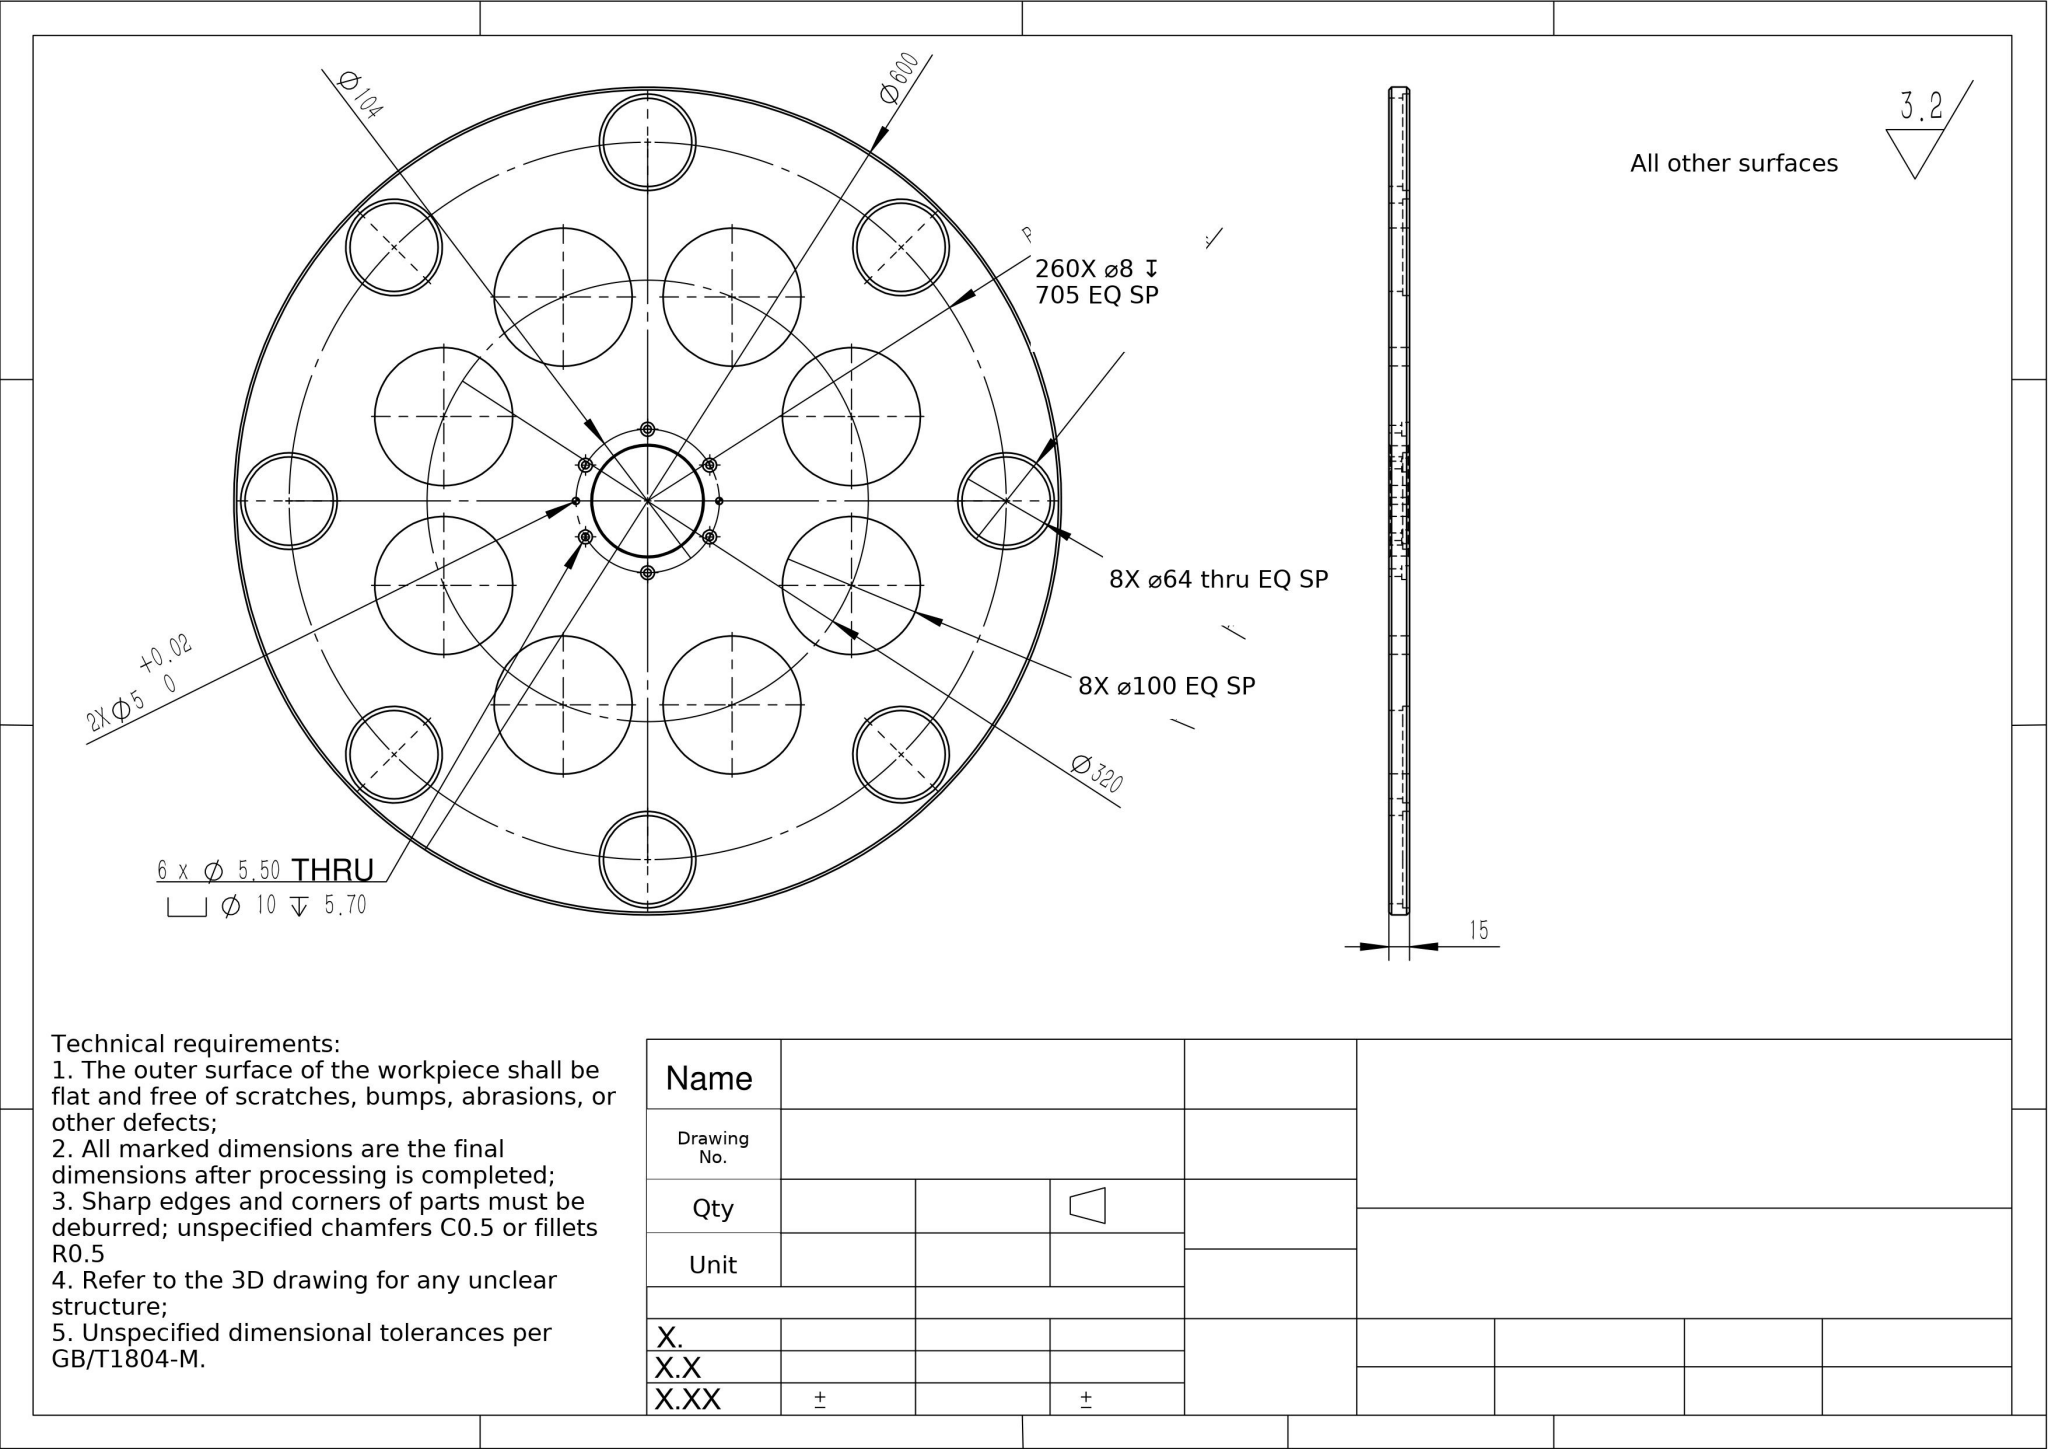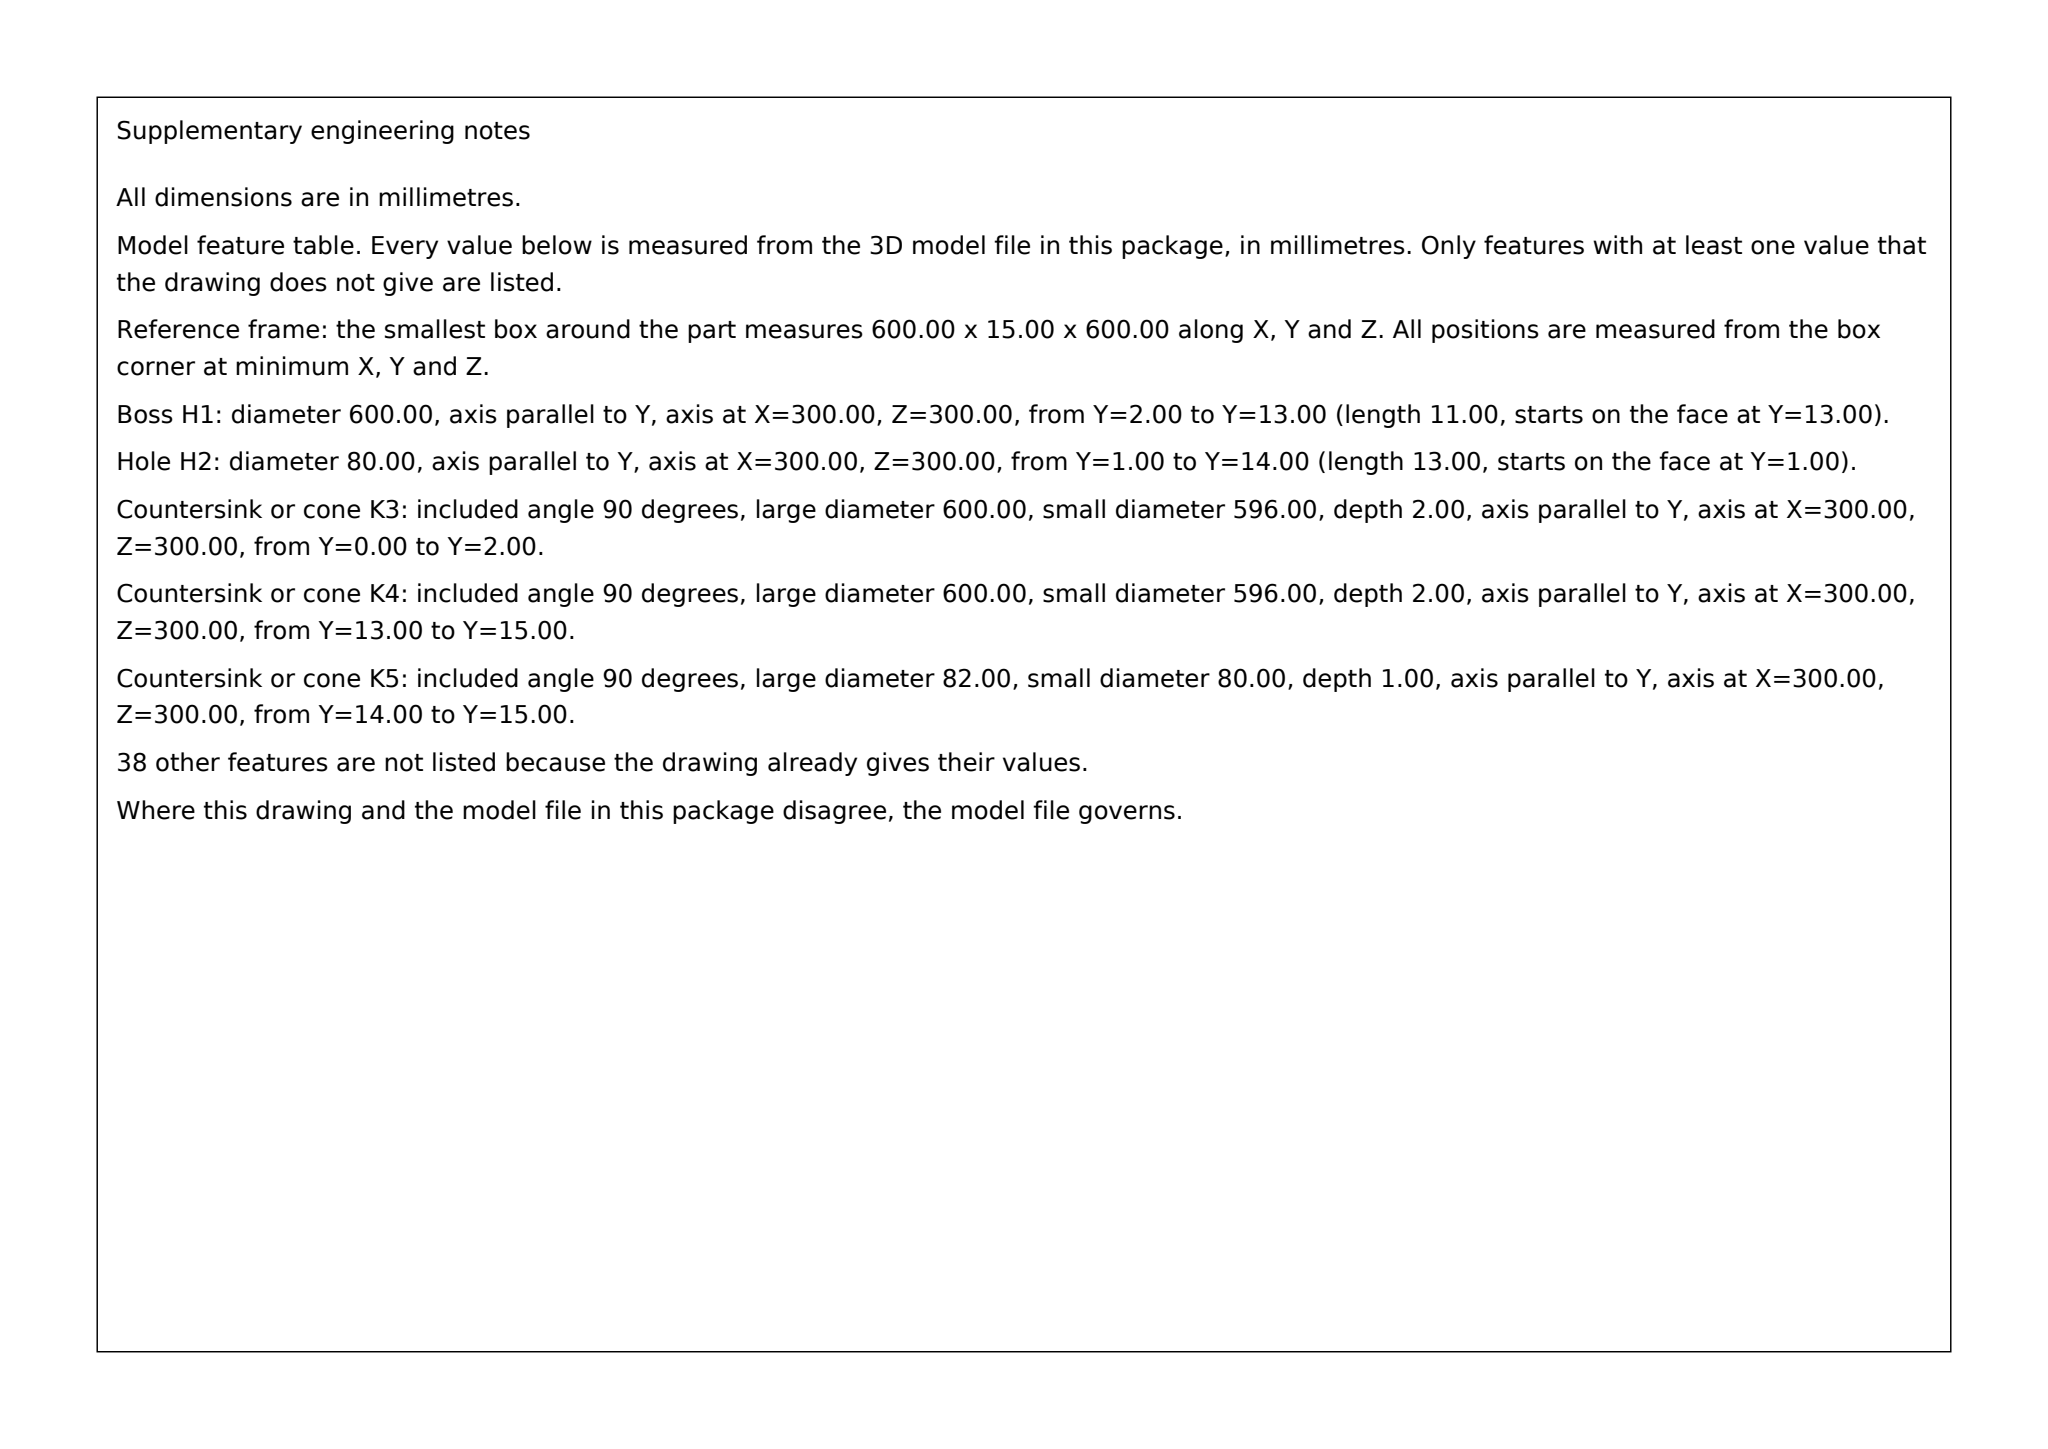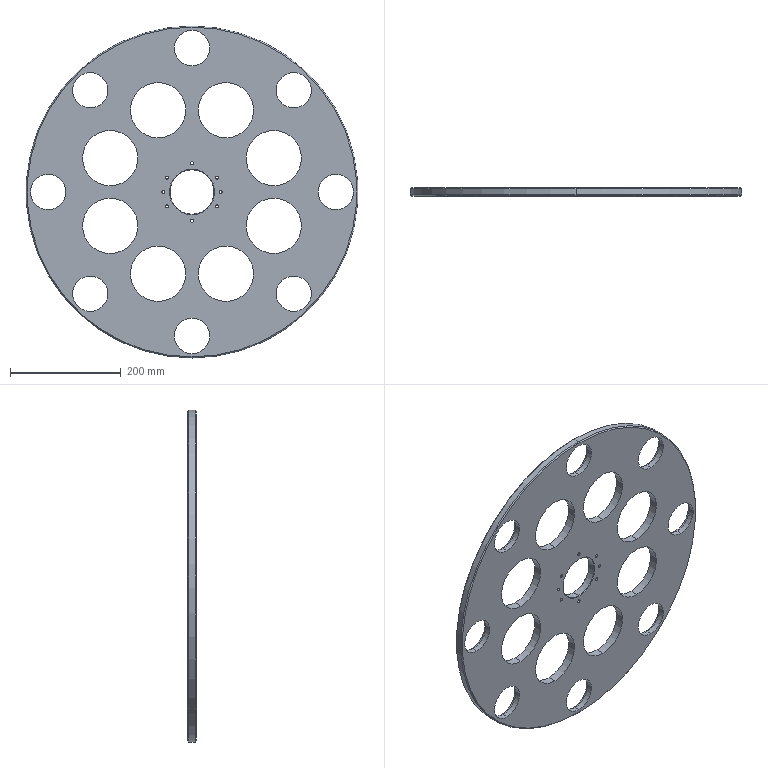Part | SolidWorks | mm | 1 solid | 104 faces | box 600 x 15 x 600 mm | volume 2799599 mm3 | cylinder 80 | plane 16 | cone 8 | commonest cylinder face diameters 100 x16 70 x16 64 x16 10 x12 5.5 x12 5 x4 80 x2 600 x2
build123d program:
from build123d import *

# Parameters (mm, degrees)
SKETCH1_R                                         = 300
SKETCH1_R_2                                       = 40
BOSS_EXTRUDE1_DEPTH                               = 15
HOLE_SIZE_ACCORDING_TO_HEXAGON_SOCKET_D           = 5.5
HOLE_SIZE_ACCORDING_TO_HEXAGON_SOCKET_CBORE_D     = 10
HOLE_SIZE_ACCORDING_TO_HEXAGON_SOCKET_CBORE_DEPTH = 5.7
SIZE_MM_DOWEL_PIN_HOLE_2_D                        = 5
CHAMFER1_SIZE                                     = 2
CHAMFER2_SIZE                                     = 1
SKETCH6_R                                         = 32
CUT_EXTRUDE1_DEPTH                                = 15
SKETCH7_R                                         = 35
CUT_EXTRUDE3_DEPTH                                = 5
CIRPATTERN1_COUNT                                 = 8
SKETCH8_R                                         = 50
CUT_EXTRUDE4_DEPTH                                = 15


with BuildPart() as part:
    # Sketch1 → Boss-Extrude1 (new body)
    with BuildSketch(Plane(origin=(0, 0, 0), x_dir=(1, 0, 0), z_dir=(0, 1, 0))):
        with Locations(Location((0, 0, 0), (0, 0, 270))):
            Circle(SKETCH1_R)
        with Locations(Location((0, 0, 0), (0, 0, 270))):
            Circle(SKETCH1_R_2, mode=Mode.SUBTRACT)
    extrude(amount=BOSS_EXTRUDE1_DEPTH)

    # Hole Size _ according to_ Hexagon Socket (through all)
    with Locations(Plane(origin=(-45.033, 15, -26), x_dir=(0, 0, 1), z_dir=(0, 1, 0))):
        with Locations((0, 0), (-26, 45.033), (0, 90.067), (52, 90.067), (78, 45.033), (52, 0)):
            CounterBoreHole(HOLE_SIZE_ACCORDING_TO_HEXAGON_SOCKET_D / 2, HOLE_SIZE_ACCORDING_TO_HEXAGON_SOCKET_CBORE_D / 2, HOLE_SIZE_ACCORDING_TO_HEXAGON_SOCKET_CBORE_DEPTH)

    # Size mm Dowel Pin Hole 2 (through all)
    with Locations(Plane(origin=(-52, 15, 0), x_dir=(0, 0, 1), z_dir=(0, 1, 0))):
        with Locations((0, 0), (0, 104)):
            Hole(SIZE_MM_DOWEL_PIN_HOLE_2_D / 2)

    # Chamfer1
    chamfer1_edges = [part.edges().sort_by_distance(p)[0] for p in [
        (0, 0, -300),
        (0, 15, -300),
    ]]
    chamfer(chamfer1_edges, length=CHAMFER1_SIZE)

    # Chamfer2
    chamfer2_edges = [part.edges().sort_by_distance(p)[0] for p in [
        (0, 0, -40),
        (0, 15, -40),
    ]]
    chamfer(chamfer2_edges, length=CHAMFER2_SIZE)

    # Sketch6 → Cut-Extrude1 (cut)
    with BuildSketch(Plane(origin=(0, 15, 0), x_dir=(1, 0, 0), z_dir=(0, 1, 0))):
        with Locations(Location((260, 0, 0), (0, 0, 270))):
            Circle(SKETCH6_R)
    cut_extrude1 = extrude(amount=-CUT_EXTRUDE1_DEPTH, mode=Mode.SUBTRACT)

    # Sketch7 → Cut-Extrude3 (cut)
    with BuildSketch(Plane(origin=(0, 15, 0), x_dir=(1, 0, 0), z_dir=(0, 1, 0))):
        with Locations(Location((260, 0, 0), (0, 0, 270))):
            Circle(SKETCH7_R)
    cut_extrude3 = extrude(amount=-CUT_EXTRUDE3_DEPTH, mode=Mode.SUBTRACT)

    # CirPattern1: Cut-Extrude1, Cut-Extrude3 ×8 about axis
    cirpattern1_axis = Axis((0, 0, 0), (0, 1, 0))
    add([cut_extrude1.rotate(cirpattern1_axis, i * 360 / CIRPATTERN1_COUNT) for i in range(1, CIRPATTERN1_COUNT)], mode=Mode.SUBTRACT)
    add([cut_extrude3.rotate(cirpattern1_axis, i * 360 / CIRPATTERN1_COUNT) for i in range(1, CIRPATTERN1_COUNT)], mode=Mode.SUBTRACT)

    # Sketch8 → Cut-Extrude4 (cut)
    with BuildSketch(Plane(origin=(0, 15, 0), x_dir=(1, 0, 0), z_dir=(0, 1, 0))):
        with Locations(Location((147.821, 61.229, 0), (0, 0, 270))):
            Circle(SKETCH8_R)
        with Locations(Location((147.821, -61.229, 0), (0, 0, 270))):
            Circle(SKETCH8_R)
        with Locations(Location((61.229, -147.821, 0), (0, 0, 270))):
            Circle(SKETCH8_R)
        with Locations(Location((-61.229, -147.821, 0), (0, 0, 270))):
            Circle(SKETCH8_R)
        with Locations(Location((-147.821, -61.229, 0), (0, 0, 270))):
            Circle(SKETCH8_R)
        with Locations(Location((-147.821, 61.229, 0), (0, 0, 270))):
            Circle(SKETCH8_R)
        with Locations(Location((-61.229, 147.821, 0), (0, 0, 270))):
            Circle(SKETCH8_R)
        with Locations(Location((61.229, 147.821, 0), (0, 0, 270))):
            Circle(SKETCH8_R)
    extrude(amount=-CUT_EXTRUDE4_DEPTH, mode=Mode.SUBTRACT)


solid = part.part